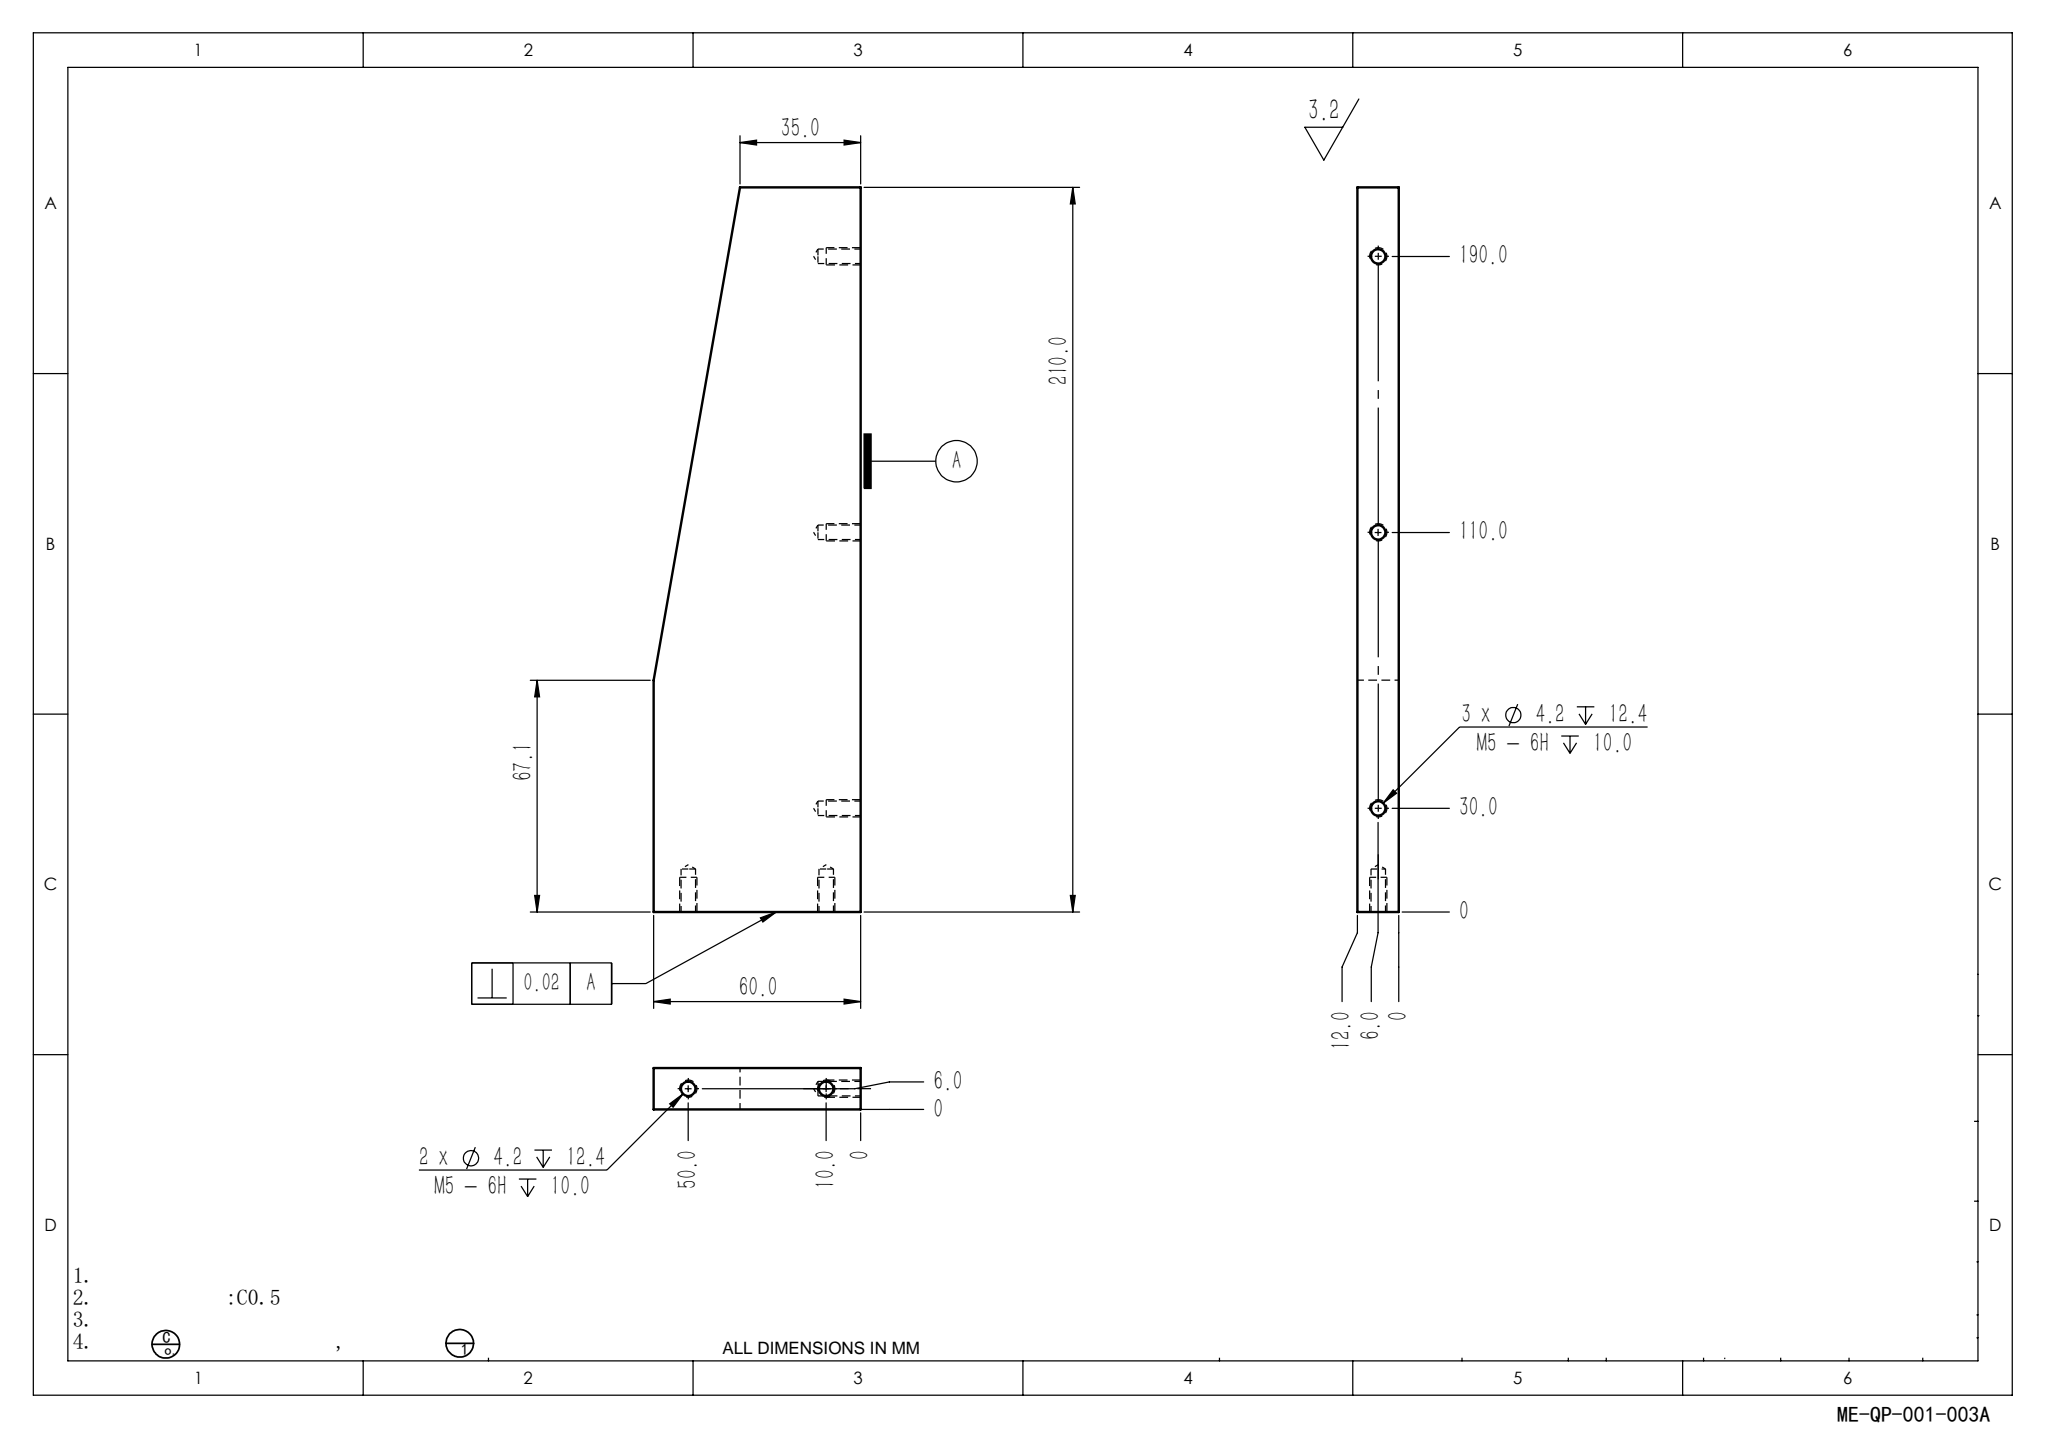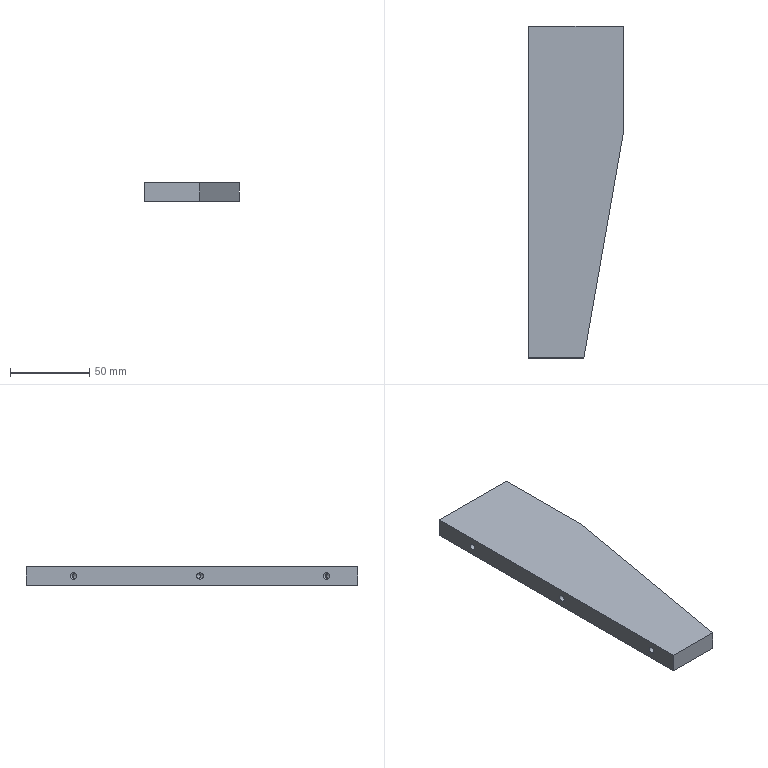Part | SolidWorks | mm | 1 solid | 27 faces | box 60 x 210 x 12 mm | volume 128883 mm3 | cylinder 10 | cone 10 | plane 7 | commonest cylinder face diameters 4.2 x10
STEP:
#1=CARTESIAN_POINT('',(-40.1,-85.,3.9));
#2=VERTEX_POINT('',#1);
#3=CARTESIAN_POINT('',(-40.1,-85.,8.1));
#4=VERTEX_POINT('',#3);
#5=CARTESIAN_POINT('',(-40.1,-85.,6.));
#6=DIRECTION('',(-1.,0.,0.));
#7=DIRECTION('',(0.,0.,1.));
#8=AXIS2_PLACEMENT_3D('',#5,#6,#7);
#9=CIRCLE('',#8,2.1);
#10=EDGE_CURVE('',#2,#4,#9,.T.);
#11=ORIENTED_EDGE('',*,*,#10,.F.);
#12=CARTESIAN_POINT('',(-52.5,-85.,3.9));
#13=VERTEX_POINT('',#12);
#14=CARTESIAN_POINT('',(-52.5,-85.,3.9));
#15=DIRECTION('',(-1.,0.,0.));
#16=VECTOR('',#15,1000.);
#17=LINE('',#14,#16);
#18=EDGE_CURVE('',#2,#13,#17,.T.);
#19=ORIENTED_EDGE('',*,*,#18,.T.);
#20=CARTESIAN_POINT('',(-52.5,-85.,8.1));
#21=VERTEX_POINT('',#20);
#22=CARTESIAN_POINT('',(-52.5,-85.,6.));
#23=DIRECTION('',(-1.,0.,0.));
#24=DIRECTION('',(0.,0.,1.));
#25=AXIS2_PLACEMENT_3D('',#22,#23,#24);
#26=CIRCLE('',#25,2.1);
#27=EDGE_CURVE('',#13,#21,#26,.T.);
#28=ORIENTED_EDGE('',*,*,#27,.T.);
#29=CARTESIAN_POINT('',(-52.5,-85.,8.1));
#30=DIRECTION('',(-1.,0.,0.));
#31=VECTOR('',#30,1000.);
#32=LINE('',#29,#31);
#33=EDGE_CURVE('',#4,#21,#32,.T.);
#34=ORIENTED_EDGE('',*,*,#33,.F.);
#35=EDGE_LOOP('',(#11,#19,#28,#34));
#36=FACE_OUTER_BOUND('',#35,.T.);
#37=CARTESIAN_POINT('',(-52.5,-85.,6.));
#38=DIRECTION('',(-1.,0.,0.));
#39=DIRECTION('',(0.,0.,1.));
#40=AXIS2_PLACEMENT_3D('',#37,#38,#39);
#41=CYLINDRICAL_SURFACE('',#40,2.1);
#42=ADVANCED_FACE('',(#36),#41,.F.);
#43=CARTESIAN_POINT('',(-38.838,-85.,6.));
#44=VERTEX_POINT('',#43);
#45=CARTESIAN_POINT('',(-40.1,-85.,8.1));
#46=DIRECTION('',(-0.515,0.,0.8572));
#47=VECTOR('',#46,1000.);
#48=LINE('',#45,#47);
#49=EDGE_CURVE('',#44,#4,#48,.T.);
#50=ORIENTED_EDGE('',*,*,#49,.F.);
#51=CARTESIAN_POINT('',(-40.1,-85.,3.9));
#52=DIRECTION('',(-0.515,0.,-0.8572));
#53=VECTOR('',#52,1000.);
#54=LINE('',#51,#53);
#55=EDGE_CURVE('',#44,#2,#54,.T.);
#56=ORIENTED_EDGE('',*,*,#55,.T.);
#57=ORIENTED_EDGE('',*,*,#10,.T.);
#58=EDGE_LOOP('',(#50,#56,#57));
#59=FACE_OUTER_BOUND('',#58,.T.);
#60=CARTESIAN_POINT('',(-40.1,-85.,6.));
#61=DIRECTION('',(-1.,0.,0.));
#62=DIRECTION('',(0.,0.,1.));
#63=AXIS2_PLACEMENT_3D('',#60,#61,#62);
#64=CONICAL_SURFACE('',#63,2.1,1.03);
#65=ADVANCED_FACE('',(#59),#64,.F.);
#66=CARTESIAN_POINT('',(-40.1,-5.,3.9));
#67=VERTEX_POINT('',#66);
#68=CARTESIAN_POINT('',(-40.1,-5.,8.1));
#69=VERTEX_POINT('',#68);
#70=CARTESIAN_POINT('',(-40.1,-5.,6.));
#71=DIRECTION('',(-1.,0.,0.));
#72=DIRECTION('',(0.,0.,1.));
#73=AXIS2_PLACEMENT_3D('',#70,#71,#72);
#74=CIRCLE('',#73,2.1);
#75=EDGE_CURVE('',#67,#69,#74,.T.);
#76=ORIENTED_EDGE('',*,*,#75,.F.);
#77=CARTESIAN_POINT('',(-52.5,-5.,3.9));
#78=VERTEX_POINT('',#77);
#79=CARTESIAN_POINT('',(-52.5,-5.,3.9));
#80=DIRECTION('',(-1.,0.,0.));
#81=VECTOR('',#80,1000.);
#82=LINE('',#79,#81);
#83=EDGE_CURVE('',#67,#78,#82,.T.);
#84=ORIENTED_EDGE('',*,*,#83,.T.);
#85=CARTESIAN_POINT('',(-52.5,-5.,8.1));
#86=VERTEX_POINT('',#85);
#87=CARTESIAN_POINT('',(-52.5,-5.,6.));
#88=DIRECTION('',(-1.,0.,0.));
#89=DIRECTION('',(0.,0.,1.));
#90=AXIS2_PLACEMENT_3D('',#87,#88,#89);
#91=CIRCLE('',#90,2.1);
#92=EDGE_CURVE('',#78,#86,#91,.T.);
#93=ORIENTED_EDGE('',*,*,#92,.T.);
#94=CARTESIAN_POINT('',(-52.5,-5.,8.1));
#95=DIRECTION('',(-1.,0.,0.));
#96=VECTOR('',#95,1000.);
#97=LINE('',#94,#96);
#98=EDGE_CURVE('',#69,#86,#97,.T.);
#99=ORIENTED_EDGE('',*,*,#98,.F.);
#100=EDGE_LOOP('',(#76,#84,#93,#99));
#101=FACE_OUTER_BOUND('',#100,.T.);
#102=CARTESIAN_POINT('',(-52.5,-5.,6.));
#103=DIRECTION('',(-1.,0.,0.));
#104=DIRECTION('',(0.,0.,1.));
#105=AXIS2_PLACEMENT_3D('',#102,#103,#104);
#106=CYLINDRICAL_SURFACE('',#105,2.1);
#107=ADVANCED_FACE('',(#101),#106,.F.);
#108=CARTESIAN_POINT('',(-38.838,-5.,6.));
#109=VERTEX_POINT('',#108);
#110=CARTESIAN_POINT('',(-40.1,-5.,8.1));
#111=DIRECTION('',(-0.515,0.,0.8572));
#112=VECTOR('',#111,1000.);
#113=LINE('',#110,#112);
#114=EDGE_CURVE('',#109,#69,#113,.T.);
#115=ORIENTED_EDGE('',*,*,#114,.F.);
#116=CARTESIAN_POINT('',(-40.1,-5.,3.9));
#117=DIRECTION('',(-0.515,0.,-0.8572));
#118=VECTOR('',#117,1000.);
#119=LINE('',#116,#118);
#120=EDGE_CURVE('',#109,#67,#119,.T.);
#121=ORIENTED_EDGE('',*,*,#120,.T.);
#122=ORIENTED_EDGE('',*,*,#75,.T.);
#123=EDGE_LOOP('',(#115,#121,#122));
#124=FACE_OUTER_BOUND('',#123,.T.);
#125=CARTESIAN_POINT('',(-40.1,-5.,6.));
#126=DIRECTION('',(-1.,0.,0.));
#127=DIRECTION('',(0.,0.,1.));
#128=AXIS2_PLACEMENT_3D('',#125,#126,#127);
#129=CONICAL_SURFACE('',#128,2.1,1.03);
#130=ADVANCED_FACE('',(#124),#129,.F.);
#131=CARTESIAN_POINT('',(-40.1,75.,3.9));
#132=VERTEX_POINT('',#131);
#133=CARTESIAN_POINT('',(-40.1,75.,8.1));
#134=VERTEX_POINT('',#133);
#135=CARTESIAN_POINT('',(-40.1,75.,6.));
#136=DIRECTION('',(-1.,0.,0.));
#137=DIRECTION('',(0.,0.,1.));
#138=AXIS2_PLACEMENT_3D('',#135,#136,#137);
#139=CIRCLE('',#138,2.1);
#140=EDGE_CURVE('',#132,#134,#139,.T.);
#141=ORIENTED_EDGE('',*,*,#140,.F.);
#142=CARTESIAN_POINT('',(-52.5,75.,3.9));
#143=VERTEX_POINT('',#142);
#144=CARTESIAN_POINT('',(-52.5,75.,3.9));
#145=DIRECTION('',(-1.,0.,0.));
#146=VECTOR('',#145,1000.);
#147=LINE('',#144,#146);
#148=EDGE_CURVE('',#132,#143,#147,.T.);
#149=ORIENTED_EDGE('',*,*,#148,.T.);
#150=CARTESIAN_POINT('',(-52.5,75.,8.1));
#151=VERTEX_POINT('',#150);
#152=CARTESIAN_POINT('',(-52.5,75.,6.));
#153=DIRECTION('',(-1.,0.,0.));
#154=DIRECTION('',(0.,0.,1.));
#155=AXIS2_PLACEMENT_3D('',#152,#153,#154);
#156=CIRCLE('',#155,2.1);
#157=EDGE_CURVE('',#143,#151,#156,.T.);
#158=ORIENTED_EDGE('',*,*,#157,.T.);
#159=CARTESIAN_POINT('',(-52.5,75.,8.1));
#160=DIRECTION('',(-1.,0.,0.));
#161=VECTOR('',#160,1000.);
#162=LINE('',#159,#161);
#163=EDGE_CURVE('',#134,#151,#162,.T.);
#164=ORIENTED_EDGE('',*,*,#163,.F.);
#165=EDGE_LOOP('',(#141,#149,#158,#164));
#166=FACE_OUTER_BOUND('',#165,.T.);
#167=CARTESIAN_POINT('',(-52.5,75.,6.));
#168=DIRECTION('',(-1.,0.,0.));
#169=DIRECTION('',(0.,0.,1.));
#170=AXIS2_PLACEMENT_3D('',#167,#168,#169);
#171=CYLINDRICAL_SURFACE('',#170,2.1);
#172=ADVANCED_FACE('',(#166),#171,.F.);
#173=CARTESIAN_POINT('',(-38.838,75.,6.));
#174=VERTEX_POINT('',#173);
#175=CARTESIAN_POINT('',(-40.1,75.,8.1));
#176=DIRECTION('',(-0.515,0.,0.8572));
#177=VECTOR('',#176,1000.);
#178=LINE('',#175,#177);
#179=EDGE_CURVE('',#174,#134,#178,.T.);
#180=ORIENTED_EDGE('',*,*,#179,.F.);
#181=CARTESIAN_POINT('',(-40.1,75.,3.9));
#182=DIRECTION('',(-0.515,0.,-0.8572));
#183=VECTOR('',#182,1000.);
#184=LINE('',#181,#183);
#185=EDGE_CURVE('',#174,#132,#184,.T.);
#186=ORIENTED_EDGE('',*,*,#185,.T.);
#187=ORIENTED_EDGE('',*,*,#140,.T.);
#188=EDGE_LOOP('',(#180,#186,#187));
#189=FACE_OUTER_BOUND('',#188,.T.);
#190=CARTESIAN_POINT('',(-40.1,75.,6.));
#191=DIRECTION('',(-1.,0.,0.));
#192=DIRECTION('',(0.,0.,1.));
#193=AXIS2_PLACEMENT_3D('',#190,#191,#192);
#194=CONICAL_SURFACE('',#193,2.1,1.03);
#195=ADVANCED_FACE('',(#189),#194,.F.);
#196=CARTESIAN_POINT('',(-42.5,92.6,3.9));
#197=VERTEX_POINT('',#196);
#198=CARTESIAN_POINT('',(-42.5,92.6,8.1));
#199=VERTEX_POINT('',#198);
#200=CARTESIAN_POINT('',(-42.5,92.6,6.));
#201=DIRECTION('',(0.,1.,0.));
#202=DIRECTION('',(0.,0.,1.));
#203=AXIS2_PLACEMENT_3D('',#200,#201,#202);
#204=CIRCLE('',#203,2.1);
#205=EDGE_CURVE('',#197,#199,#204,.T.);
#206=ORIENTED_EDGE('',*,*,#205,.F.);
#207=CARTESIAN_POINT('',(-42.5,105.,3.9));
#208=VERTEX_POINT('',#207);
#209=CARTESIAN_POINT('',(-42.5,105.,3.9));
#210=DIRECTION('',(0.,1.,0.));
#211=VECTOR('',#210,1000.);
#212=LINE('',#209,#211);
#213=EDGE_CURVE('',#197,#208,#212,.T.);
#214=ORIENTED_EDGE('',*,*,#213,.T.);
#215=CARTESIAN_POINT('',(-42.5,105.,8.1));
#216=VERTEX_POINT('',#215);
#217=CARTESIAN_POINT('',(-42.5,105.,6.));
#218=DIRECTION('',(0.,1.,0.));
#219=DIRECTION('',(0.,0.,1.));
#220=AXIS2_PLACEMENT_3D('',#217,#218,#219);
#221=CIRCLE('',#220,2.1);
#222=EDGE_CURVE('',#208,#216,#221,.T.);
#223=ORIENTED_EDGE('',*,*,#222,.T.);
#224=CARTESIAN_POINT('',(-42.5,105.,8.1));
#225=DIRECTION('',(0.,1.,0.));
#226=VECTOR('',#225,1000.);
#227=LINE('',#224,#226);
#228=EDGE_CURVE('',#199,#216,#227,.T.);
#229=ORIENTED_EDGE('',*,*,#228,.F.);
#230=EDGE_LOOP('',(#206,#214,#223,#229));
#231=FACE_OUTER_BOUND('',#230,.T.);
#232=CARTESIAN_POINT('',(-42.5,105.,6.));
#233=DIRECTION('',(0.,1.,0.));
#234=DIRECTION('',(0.,0.,1.));
#235=AXIS2_PLACEMENT_3D('',#232,#233,#234);
#236=CYLINDRICAL_SURFACE('',#235,2.1);
#237=ADVANCED_FACE('',(#231),#236,.F.);
#238=CARTESIAN_POINT('',(-42.5,91.338,6.));
#239=VERTEX_POINT('',#238);
#240=CARTESIAN_POINT('',(-42.5,92.6,8.1));
#241=DIRECTION('',(0.,0.515,0.8572));
#242=VECTOR('',#241,1000.);
#243=LINE('',#240,#242);
#244=EDGE_CURVE('',#239,#199,#243,.T.);
#245=ORIENTED_EDGE('',*,*,#244,.F.);
#246=CARTESIAN_POINT('',(-42.5,92.6,3.9));
#247=DIRECTION('',(0.,0.515,-0.8572));
#248=VECTOR('',#247,1000.);
#249=LINE('',#246,#248);
#250=EDGE_CURVE('',#239,#197,#249,.T.);
#251=ORIENTED_EDGE('',*,*,#250,.T.);
#252=ORIENTED_EDGE('',*,*,#205,.T.);
#253=EDGE_LOOP('',(#245,#251,#252));
#254=FACE_OUTER_BOUND('',#253,.T.);
#255=CARTESIAN_POINT('',(-42.5,92.6,6.));
#256=DIRECTION('',(0.,1.,0.));
#257=DIRECTION('',(0.,0.,1.));
#258=AXIS2_PLACEMENT_3D('',#255,#256,#257);
#259=CONICAL_SURFACE('',#258,2.1,1.03);
#260=ADVANCED_FACE('',(#254),#259,.F.);
#261=CARTESIAN_POINT('',(-2.5,92.6,3.9));
#262=VERTEX_POINT('',#261);
#263=CARTESIAN_POINT('',(-2.5,92.6,8.1));
#264=VERTEX_POINT('',#263);
#265=CARTESIAN_POINT('',(-2.5,92.6,6.));
#266=DIRECTION('',(0.,1.,0.));
#267=DIRECTION('',(0.,0.,1.));
#268=AXIS2_PLACEMENT_3D('',#265,#266,#267);
#269=CIRCLE('',#268,2.1);
#270=EDGE_CURVE('',#262,#264,#269,.T.);
#271=ORIENTED_EDGE('',*,*,#270,.F.);
#272=CARTESIAN_POINT('',(-2.5,105.,3.9));
#273=VERTEX_POINT('',#272);
#274=CARTESIAN_POINT('',(-2.5,105.,3.9));
#275=DIRECTION('',(0.,1.,0.));
#276=VECTOR('',#275,1000.);
#277=LINE('',#274,#276);
#278=EDGE_CURVE('',#262,#273,#277,.T.);
#279=ORIENTED_EDGE('',*,*,#278,.T.);
#280=CARTESIAN_POINT('',(-2.5,105.,8.1));
#281=VERTEX_POINT('',#280);
#282=CARTESIAN_POINT('',(-2.5,105.,6.));
#283=DIRECTION('',(0.,1.,0.));
#284=DIRECTION('',(0.,0.,1.));
#285=AXIS2_PLACEMENT_3D('',#282,#283,#284);
#286=CIRCLE('',#285,2.1);
#287=EDGE_CURVE('',#273,#281,#286,.T.);
#288=ORIENTED_EDGE('',*,*,#287,.T.);
#289=CARTESIAN_POINT('',(-2.5,105.,8.1));
#290=DIRECTION('',(0.,1.,0.));
#291=VECTOR('',#290,1000.);
#292=LINE('',#289,#291);
#293=EDGE_CURVE('',#264,#281,#292,.T.);
#294=ORIENTED_EDGE('',*,*,#293,.F.);
#295=EDGE_LOOP('',(#271,#279,#288,#294));
#296=FACE_OUTER_BOUND('',#295,.T.);
#297=CARTESIAN_POINT('',(-2.5,105.,6.));
#298=DIRECTION('',(0.,1.,0.));
#299=DIRECTION('',(0.,0.,1.));
#300=AXIS2_PLACEMENT_3D('',#297,#298,#299);
#301=CYLINDRICAL_SURFACE('',#300,2.1);
#302=ADVANCED_FACE('',(#296),#301,.F.);
#303=CARTESIAN_POINT('',(-2.5,91.338,6.));
#304=VERTEX_POINT('',#303);
#305=CARTESIAN_POINT('',(-2.5,92.6,8.1));
#306=DIRECTION('',(0.,0.515,0.8572));
#307=VECTOR('',#306,1000.);
#308=LINE('',#305,#307);
#309=EDGE_CURVE('',#304,#264,#308,.T.);
#310=ORIENTED_EDGE('',*,*,#309,.F.);
#311=CARTESIAN_POINT('',(-2.5,92.6,3.9));
#312=DIRECTION('',(0.,0.515,-0.8572));
#313=VECTOR('',#312,1000.);
#314=LINE('',#311,#313);
#315=EDGE_CURVE('',#304,#262,#314,.T.);
#316=ORIENTED_EDGE('',*,*,#315,.T.);
#317=ORIENTED_EDGE('',*,*,#270,.T.);
#318=EDGE_LOOP('',(#310,#316,#317));
#319=FACE_OUTER_BOUND('',#318,.T.);
#320=CARTESIAN_POINT('',(-2.5,92.6,6.));
#321=DIRECTION('',(0.,1.,0.));
#322=DIRECTION('',(0.,0.,1.));
#323=AXIS2_PLACEMENT_3D('',#320,#321,#322);
#324=CONICAL_SURFACE('',#323,2.1,1.03);
#325=ADVANCED_FACE('',(#319),#324,.F.);
#326=CARTESIAN_POINT('',(-52.5,-85.,6.));
#327=DIRECTION('',(-1.,0.,0.));
#328=DIRECTION('',(0.,0.,1.));
#329=AXIS2_PLACEMENT_3D('',#326,#327,#328);
#330=CIRCLE('',#329,2.1);
#331=EDGE_CURVE('',#21,#13,#330,.T.);
#332=ORIENTED_EDGE('',*,*,#331,.F.);
#333=ORIENTED_EDGE('',*,*,#27,.F.);
#334=EDGE_LOOP('',(#332,#333));
#335=FACE_BOUND('',#334,.T.);
#336=CARTESIAN_POINT('',(-52.5,-5.,6.));
#337=DIRECTION('',(-1.,0.,0.));
#338=DIRECTION('',(0.,0.,1.));
#339=AXIS2_PLACEMENT_3D('',#336,#337,#338);
#340=CIRCLE('',#339,2.1);
#341=EDGE_CURVE('',#86,#78,#340,.T.);
#342=ORIENTED_EDGE('',*,*,#341,.F.);
#343=ORIENTED_EDGE('',*,*,#92,.F.);
#344=EDGE_LOOP('',(#342,#343));
#345=FACE_BOUND('',#344,.T.);
#346=CARTESIAN_POINT('',(-52.5,75.,6.));
#347=DIRECTION('',(-1.,0.,0.));
#348=DIRECTION('',(0.,0.,1.));
#349=AXIS2_PLACEMENT_3D('',#346,#347,#348);
#350=CIRCLE('',#349,2.1);
#351=EDGE_CURVE('',#151,#143,#350,.T.);
#352=ORIENTED_EDGE('',*,*,#351,.F.);
#353=ORIENTED_EDGE('',*,*,#157,.F.);
#354=EDGE_LOOP('',(#352,#353));
#355=FACE_BOUND('',#354,.T.);
#356=CARTESIAN_POINT('',(-52.5,105.,0.));
#357=VERTEX_POINT('',#356);
#358=CARTESIAN_POINT('',(-52.5,-105.,0.));
#359=VERTEX_POINT('',#358);
#360=CARTESIAN_POINT('',(-52.5,-105.,0.));
#361=DIRECTION('',(0.,-1.,0.));
#362=VECTOR('',#361,1000.);
#363=LINE('',#360,#362);
#364=EDGE_CURVE('',#357,#359,#363,.T.);
#365=ORIENTED_EDGE('',*,*,#364,.T.);
#366=CARTESIAN_POINT('',(-52.5,-105.,12.));
#367=VERTEX_POINT('',#366);
#368=CARTESIAN_POINT('',(-52.5,-105.,12.));
#369=DIRECTION('',(0.,0.,-1.));
#370=VECTOR('',#369,1000.);
#371=LINE('',#368,#370);
#372=EDGE_CURVE('',#367,#359,#371,.T.);
#373=ORIENTED_EDGE('',*,*,#372,.F.);
#374=CARTESIAN_POINT('',(-52.5,105.,12.));
#375=VERTEX_POINT('',#374);
#376=CARTESIAN_POINT('',(-52.5,-105.,12.));
#377=DIRECTION('',(0.,-1.,0.));
#378=VECTOR('',#377,1000.);
#379=LINE('',#376,#378);
#380=EDGE_CURVE('',#375,#367,#379,.T.);
#381=ORIENTED_EDGE('',*,*,#380,.F.);
#382=CARTESIAN_POINT('',(-52.5,105.,12.));
#383=DIRECTION('',(0.,0.,-1.));
#384=VECTOR('',#383,1000.);
#385=LINE('',#382,#384);
#386=EDGE_CURVE('',#375,#357,#385,.T.);
#387=ORIENTED_EDGE('',*,*,#386,.T.);
#388=EDGE_LOOP('',(#365,#373,#381,#387));
#389=FACE_OUTER_BOUND('',#388,.T.);
#390=CARTESIAN_POINT('',(-52.5,-105.,12.));
#391=DIRECTION('',(1.,0.,0.));
#392=DIRECTION('',(0.,0.,-1.));
#393=AXIS2_PLACEMENT_3D('',#390,#391,#392);
#394=PLANE('',#393);
#395=ADVANCED_FACE('',(#335,#345,#355,#389),#394,.F.);
#396=CARTESIAN_POINT('',(-17.5,-105.,0.));
#397=VERTEX_POINT('',#396);
#398=CARTESIAN_POINT('',(52.5,-105.,0.));
#399=DIRECTION('',(1.,0.,0.));
#400=VECTOR('',#399,1000.);
#401=LINE('',#398,#400);
#402=EDGE_CURVE('',#359,#397,#401,.T.);
#403=ORIENTED_EDGE('',*,*,#402,.T.);
#404=CARTESIAN_POINT('',(-17.5,-105.,12.));
#405=VERTEX_POINT('',#404);
#406=CARTESIAN_POINT('',(-17.5,-105.,12.));
#407=DIRECTION('',(0.,0.,1.));
#408=VECTOR('',#407,1000.);
#409=LINE('',#406,#408);
#410=EDGE_CURVE('',#397,#405,#409,.T.);
#411=ORIENTED_EDGE('',*,*,#410,.T.);
#412=CARTESIAN_POINT('',(52.5,-105.,12.));
#413=DIRECTION('',(1.,0.,0.));
#414=VECTOR('',#413,1000.);
#415=LINE('',#412,#414);
#416=EDGE_CURVE('',#367,#405,#415,.T.);
#417=ORIENTED_EDGE('',*,*,#416,.F.);
#418=ORIENTED_EDGE('',*,*,#372,.T.);
#419=EDGE_LOOP('',(#403,#411,#417,#418));
#420=FACE_OUTER_BOUND('',#419,.T.);
#421=CARTESIAN_POINT('',(52.5,-105.,12.));
#422=DIRECTION('',(-0.,1.,0.));
#423=DIRECTION('',(-1.,-0.,0.));
#424=AXIS2_PLACEMENT_3D('',#421,#422,#423);
#425=PLANE('',#424);
#426=ADVANCED_FACE('',(#420),#425,.F.);
#427=CARTESIAN_POINT('',(-42.5,105.,6.));
#428=DIRECTION('',(0.,1.,0.));
#429=DIRECTION('',(0.,0.,1.));
#430=AXIS2_PLACEMENT_3D('',#427,#428,#429);
#431=CIRCLE('',#430,2.1);
#432=EDGE_CURVE('',#216,#208,#431,.T.);
#433=ORIENTED_EDGE('',*,*,#432,.F.);
#434=ORIENTED_EDGE('',*,*,#222,.F.);
#435=EDGE_LOOP('',(#433,#434));
#436=FACE_BOUND('',#435,.T.);
#437=CARTESIAN_POINT('',(-2.5,105.,6.));
#438=DIRECTION('',(0.,1.,0.));
#439=DIRECTION('',(0.,0.,1.));
#440=AXIS2_PLACEMENT_3D('',#437,#438,#439);
#441=CIRCLE('',#440,2.1);
#442=EDGE_CURVE('',#281,#273,#441,.T.);
#443=ORIENTED_EDGE('',*,*,#442,.F.);
#444=ORIENTED_EDGE('',*,*,#287,.F.);
#445=EDGE_LOOP('',(#443,#444));
#446=FACE_BOUND('',#445,.T.);
#447=CARTESIAN_POINT('',(7.5,105.,12.));
#448=VERTEX_POINT('',#447);
#449=CARTESIAN_POINT('',(52.5,105.,12.));
#450=DIRECTION('',(-1.,0.,0.));
#451=VECTOR('',#450,1000.);
#452=LINE('',#449,#451);
#453=EDGE_CURVE('',#448,#375,#452,.T.);
#454=ORIENTED_EDGE('',*,*,#453,.F.);
#455=CARTESIAN_POINT('',(7.5,105.,0.));
#456=VERTEX_POINT('',#455);
#457=CARTESIAN_POINT('',(7.5,105.,12.));
#458=DIRECTION('',(0.,0.,-1.));
#459=VECTOR('',#458,1000.);
#460=LINE('',#457,#459);
#461=EDGE_CURVE('',#448,#456,#460,.T.);
#462=ORIENTED_EDGE('',*,*,#461,.T.);
#463=CARTESIAN_POINT('',(52.5,105.,0.));
#464=DIRECTION('',(-1.,0.,0.));
#465=VECTOR('',#464,1000.);
#466=LINE('',#463,#465);
#467=EDGE_CURVE('',#456,#357,#466,.T.);
#468=ORIENTED_EDGE('',*,*,#467,.T.);
#469=ORIENTED_EDGE('',*,*,#386,.F.);
#470=EDGE_LOOP('',(#454,#462,#468,#469));
#471=FACE_OUTER_BOUND('',#470,.T.);
#472=CARTESIAN_POINT('',(52.5,105.,12.));
#473=DIRECTION('',(0.,-1.,0.));
#474=DIRECTION('',(0.,0.,-1.));
#475=AXIS2_PLACEMENT_3D('',#472,#473,#474);
#476=PLANE('',#475);
#477=ADVANCED_FACE('',(#436,#446,#471),#476,.F.);
#478=CARTESIAN_POINT('',(7.5,37.857,12.));
#479=VERTEX_POINT('',#478);
#480=CARTESIAN_POINT('',(7.5,185.,12.));
#481=DIRECTION('',(0.,1.,0.));
#482=VECTOR('',#481,1000.);
#483=LINE('',#480,#482);
#484=EDGE_CURVE('',#479,#448,#483,.T.);
#485=ORIENTED_EDGE('',*,*,#484,.T.);
#486=ORIENTED_EDGE('',*,*,#453,.T.);
#487=ORIENTED_EDGE('',*,*,#380,.T.);
#488=ORIENTED_EDGE('',*,*,#416,.T.);
#489=CARTESIAN_POINT('',(0.849,-0.1486,12.));
#490=DIRECTION('',(0.1724,0.985,0.));
#491=VECTOR('',#490,1000.);
#492=LINE('',#489,#491);
#493=EDGE_CURVE('',#405,#479,#492,.T.);
#494=ORIENTED_EDGE('',*,*,#493,.T.);
#495=EDGE_LOOP('',(#485,#486,#487,#488,#494));
#496=FACE_OUTER_BOUND('',#495,.T.);
#497=CARTESIAN_POINT('',(0.,0.,12.));
#498=DIRECTION('',(0.,0.,1.));
#499=DIRECTION('',(1.,0.,0.));
#500=AXIS2_PLACEMENT_3D('',#497,#498,#499);
#501=PLANE('',#500);
#502=ADVANCED_FACE('',(#496),#501,.T.);
#503=ORIENTED_EDGE('',*,*,#467,.F.);
#504=CARTESIAN_POINT('',(7.5,37.857,0.));
#505=VERTEX_POINT('',#504);
#506=CARTESIAN_POINT('',(7.5,185.,0.));
#507=DIRECTION('',(0.,1.,0.));
#508=VECTOR('',#507,1000.);
#509=LINE('',#506,#508);
#510=EDGE_CURVE('',#505,#456,#509,.T.);
#511=ORIENTED_EDGE('',*,*,#510,.F.);
#512=CARTESIAN_POINT('',(52.5,295.,0.));
#513=DIRECTION('',(-0.1724,-0.985,0.));
#514=VECTOR('',#513,1000.);
#515=LINE('',#512,#514);
#516=EDGE_CURVE('',#505,#397,#515,.T.);
#517=ORIENTED_EDGE('',*,*,#516,.T.);
#518=ORIENTED_EDGE('',*,*,#402,.F.);
#519=ORIENTED_EDGE('',*,*,#364,.F.);
#520=EDGE_LOOP('',(#503,#511,#517,#518,#519));
#521=FACE_OUTER_BOUND('',#520,.T.);
#522=CARTESIAN_POINT('',(0.,0.,0.));
#523=DIRECTION('',(0.,0.,1.));
#524=DIRECTION('',(1.,0.,0.));
#525=AXIS2_PLACEMENT_3D('',#522,#523,#524);
#526=PLANE('',#525);
#527=ADVANCED_FACE('',(#521),#526,.F.);
#528=CARTESIAN_POINT('',(7.5,37.857,12.));
#529=DIRECTION('',(0.,0.,-1.));
#530=VECTOR('',#529,1000.);
#531=LINE('',#528,#530);
#532=EDGE_CURVE('',#479,#505,#531,.T.);
#533=ORIENTED_EDGE('',*,*,#532,.F.);
#534=ORIENTED_EDGE('',*,*,#493,.F.);
#535=ORIENTED_EDGE('',*,*,#410,.F.);
#536=ORIENTED_EDGE('',*,*,#516,.F.);
#537=EDGE_LOOP('',(#533,#534,#535,#536));
#538=FACE_OUTER_BOUND('',#537,.T.);
#539=CARTESIAN_POINT('',(52.5,295.,12.));
#540=DIRECTION('',(-0.985,0.1724,0.));
#541=DIRECTION('',(0.,0.,-1.));
#542=AXIS2_PLACEMENT_3D('',#539,#540,#541);
#543=PLANE('',#542);
#544=ADVANCED_FACE('',(#538),#543,.F.);
#545=ORIENTED_EDGE('',*,*,#315,.F.);
#546=ORIENTED_EDGE('',*,*,#309,.T.);
#547=CARTESIAN_POINT('',(-2.5,92.6,6.));
#548=DIRECTION('',(0.,1.,0.));
#549=DIRECTION('',(0.,0.,1.));
#550=AXIS2_PLACEMENT_3D('',#547,#548,#549);
#551=CIRCLE('',#550,2.1);
#552=EDGE_CURVE('',#264,#262,#551,.T.);
#553=ORIENTED_EDGE('',*,*,#552,.T.);
#554=EDGE_LOOP('',(#545,#546,#553));
#555=FACE_OUTER_BOUND('',#554,.T.);
#556=CARTESIAN_POINT('',(-2.5,92.6,6.));
#557=DIRECTION('',(0.,1.,0.));
#558=DIRECTION('',(0.,0.,1.));
#559=AXIS2_PLACEMENT_3D('',#556,#557,#558);
#560=CONICAL_SURFACE('',#559,2.1,1.03);
#561=ADVANCED_FACE('',(#555),#560,.F.);
#562=ORIENTED_EDGE('',*,*,#278,.F.);
#563=ORIENTED_EDGE('',*,*,#552,.F.);
#564=ORIENTED_EDGE('',*,*,#293,.T.);
#565=ORIENTED_EDGE('',*,*,#442,.T.);
#566=EDGE_LOOP('',(#562,#563,#564,#565));
#567=FACE_OUTER_BOUND('',#566,.T.);
#568=CARTESIAN_POINT('',(-2.5,105.,6.));
#569=DIRECTION('',(0.,1.,0.));
#570=DIRECTION('',(0.,0.,1.));
#571=AXIS2_PLACEMENT_3D('',#568,#569,#570);
#572=CYLINDRICAL_SURFACE('',#571,2.1);
#573=ADVANCED_FACE('',(#567),#572,.F.);
#574=ORIENTED_EDGE('',*,*,#250,.F.);
#575=ORIENTED_EDGE('',*,*,#244,.T.);
#576=CARTESIAN_POINT('',(-42.5,92.6,6.));
#577=DIRECTION('',(0.,1.,0.));
#578=DIRECTION('',(0.,0.,1.));
#579=AXIS2_PLACEMENT_3D('',#576,#577,#578);
#580=CIRCLE('',#579,2.1);
#581=EDGE_CURVE('',#199,#197,#580,.T.);
#582=ORIENTED_EDGE('',*,*,#581,.T.);
#583=EDGE_LOOP('',(#574,#575,#582));
#584=FACE_OUTER_BOUND('',#583,.T.);
#585=CARTESIAN_POINT('',(-42.5,92.6,6.));
#586=DIRECTION('',(0.,1.,0.));
#587=DIRECTION('',(0.,0.,1.));
#588=AXIS2_PLACEMENT_3D('',#585,#586,#587);
#589=CONICAL_SURFACE('',#588,2.1,1.03);
#590=ADVANCED_FACE('',(#584),#589,.F.);
#591=ORIENTED_EDGE('',*,*,#213,.F.);
#592=ORIENTED_EDGE('',*,*,#581,.F.);
#593=ORIENTED_EDGE('',*,*,#228,.T.);
#594=ORIENTED_EDGE('',*,*,#432,.T.);
#595=EDGE_LOOP('',(#591,#592,#593,#594));
#596=FACE_OUTER_BOUND('',#595,.T.);
#597=CARTESIAN_POINT('',(-42.5,105.,6.));
#598=DIRECTION('',(0.,1.,0.));
#599=DIRECTION('',(0.,0.,1.));
#600=AXIS2_PLACEMENT_3D('',#597,#598,#599);
#601=CYLINDRICAL_SURFACE('',#600,2.1);
#602=ADVANCED_FACE('',(#596),#601,.F.);
#603=ORIENTED_EDGE('',*,*,#185,.F.);
#604=ORIENTED_EDGE('',*,*,#179,.T.);
#605=CARTESIAN_POINT('',(-40.1,75.,6.));
#606=DIRECTION('',(-1.,0.,0.));
#607=DIRECTION('',(0.,0.,1.));
#608=AXIS2_PLACEMENT_3D('',#605,#606,#607);
#609=CIRCLE('',#608,2.1);
#610=EDGE_CURVE('',#134,#132,#609,.T.);
#611=ORIENTED_EDGE('',*,*,#610,.T.);
#612=EDGE_LOOP('',(#603,#604,#611));
#613=FACE_OUTER_BOUND('',#612,.T.);
#614=CARTESIAN_POINT('',(-40.1,75.,6.));
#615=DIRECTION('',(-1.,0.,0.));
#616=DIRECTION('',(0.,0.,1.));
#617=AXIS2_PLACEMENT_3D('',#614,#615,#616);
#618=CONICAL_SURFACE('',#617,2.1,1.03);
#619=ADVANCED_FACE('',(#613),#618,.F.);
#620=ORIENTED_EDGE('',*,*,#148,.F.);
#621=ORIENTED_EDGE('',*,*,#610,.F.);
#622=ORIENTED_EDGE('',*,*,#163,.T.);
#623=ORIENTED_EDGE('',*,*,#351,.T.);
#624=EDGE_LOOP('',(#620,#621,#622,#623));
#625=FACE_OUTER_BOUND('',#624,.T.);
#626=CARTESIAN_POINT('',(-52.5,75.,6.));
#627=DIRECTION('',(-1.,0.,0.));
#628=DIRECTION('',(0.,0.,1.));
#629=AXIS2_PLACEMENT_3D('',#626,#627,#628);
#630=CYLINDRICAL_SURFACE('',#629,2.1);
#631=ADVANCED_FACE('',(#625),#630,.F.);
#632=ORIENTED_EDGE('',*,*,#120,.F.);
#633=ORIENTED_EDGE('',*,*,#114,.T.);
#634=CARTESIAN_POINT('',(-40.1,-5.,6.));
#635=DIRECTION('',(-1.,0.,0.));
#636=DIRECTION('',(0.,0.,1.));
#637=AXIS2_PLACEMENT_3D('',#634,#635,#636);
#638=CIRCLE('',#637,2.1);
#639=EDGE_CURVE('',#69,#67,#638,.T.);
#640=ORIENTED_EDGE('',*,*,#639,.T.);
#641=EDGE_LOOP('',(#632,#633,#640));
#642=FACE_OUTER_BOUND('',#641,.T.);
#643=CARTESIAN_POINT('',(-40.1,-5.,6.));
#644=DIRECTION('',(-1.,0.,0.));
#645=DIRECTION('',(0.,0.,1.));
#646=AXIS2_PLACEMENT_3D('',#643,#644,#645);
#647=CONICAL_SURFACE('',#646,2.1,1.03);
#648=ADVANCED_FACE('',(#642),#647,.F.);
#649=ORIENTED_EDGE('',*,*,#83,.F.);
#650=ORIENTED_EDGE('',*,*,#639,.F.);
#651=ORIENTED_EDGE('',*,*,#98,.T.);
#652=ORIENTED_EDGE('',*,*,#341,.T.);
#653=EDGE_LOOP('',(#649,#650,#651,#652));
#654=FACE_OUTER_BOUND('',#653,.T.);
#655=CARTESIAN_POINT('',(-52.5,-5.,6.));
#656=DIRECTION('',(-1.,0.,0.));
#657=DIRECTION('',(0.,0.,1.));
#658=AXIS2_PLACEMENT_3D('',#655,#656,#657);
#659=CYLINDRICAL_SURFACE('',#658,2.1);
#660=ADVANCED_FACE('',(#654),#659,.F.);
#661=ORIENTED_EDGE('',*,*,#55,.F.);
#662=ORIENTED_EDGE('',*,*,#49,.T.);
#663=CARTESIAN_POINT('',(-40.1,-85.,6.));
#664=DIRECTION('',(-1.,0.,0.));
#665=DIRECTION('',(0.,0.,1.));
#666=AXIS2_PLACEMENT_3D('',#663,#664,#665);
#667=CIRCLE('',#666,2.1);
#668=EDGE_CURVE('',#4,#2,#667,.T.);
#669=ORIENTED_EDGE('',*,*,#668,.T.);
#670=EDGE_LOOP('',(#661,#662,#669));
#671=FACE_OUTER_BOUND('',#670,.T.);
#672=CARTESIAN_POINT('',(-40.1,-85.,6.));
#673=DIRECTION('',(-1.,0.,0.));
#674=DIRECTION('',(0.,0.,1.));
#675=AXIS2_PLACEMENT_3D('',#672,#673,#674);
#676=CONICAL_SURFACE('',#675,2.1,1.03);
#677=ADVANCED_FACE('',(#671),#676,.F.);
#678=ORIENTED_EDGE('',*,*,#18,.F.);
#679=ORIENTED_EDGE('',*,*,#668,.F.);
#680=ORIENTED_EDGE('',*,*,#33,.T.);
#681=ORIENTED_EDGE('',*,*,#331,.T.);
#682=EDGE_LOOP('',(#678,#679,#680,#681));
#683=FACE_OUTER_BOUND('',#682,.T.);
#684=CARTESIAN_POINT('',(-52.5,-85.,6.));
#685=DIRECTION('',(-1.,0.,0.));
#686=DIRECTION('',(0.,0.,1.));
#687=AXIS2_PLACEMENT_3D('',#684,#685,#686);
#688=CYLINDRICAL_SURFACE('',#687,2.1);
#689=ADVANCED_FACE('',(#683),#688,.F.);
#690=ORIENTED_EDGE('',*,*,#484,.F.);
#691=ORIENTED_EDGE('',*,*,#532,.T.);
#692=ORIENTED_EDGE('',*,*,#510,.T.);
#693=ORIENTED_EDGE('',*,*,#461,.F.);
#694=EDGE_LOOP('',(#690,#691,#692,#693));
#695=FACE_OUTER_BOUND('',#694,.T.);
#696=CARTESIAN_POINT('',(7.5,185.,12.));
#697=DIRECTION('',(-1.,0.,0.));
#698=DIRECTION('',(0.,0.,1.));
#699=AXIS2_PLACEMENT_3D('',#696,#697,#698);
#700=PLANE('',#699);
#701=ADVANCED_FACE('',(#695),#700,.F.);
#702=CLOSED_SHELL('',(#42,#65,#107,#130,#172,#195,#237,#260,#302,#325,#395,#426,#477,#502,#527,#544,#561,#573,#590,#602,#619,#631,#648,#660,#677,#689,#701));
#703=MANIFOLD_SOLID_BREP('',#702);
#704=CARTESIAN_POINT('',(0.,0.,0.));
#705=DIRECTION('',(0.,0.,1.));
#706=DIRECTION('',(1.,0.,0.));
#707=AXIS2_PLACEMENT_3D('',#704,#705,#706);
#708=(LENGTH_UNIT()NAMED_UNIT(*)SI_UNIT(.MILLI.,.METRE.));
#709=UNCERTAINTY_MEASURE_WITH_UNIT(LENGTH_MEASURE(0.00001),#708,'','');
#710=(NAMED_UNIT(*)PLANE_ANGLE_UNIT()SI_UNIT($,.RADIAN.));
#711=(NAMED_UNIT(*)SI_UNIT($,.STERADIAN.)SOLID_ANGLE_UNIT());
#712=(GEOMETRIC_REPRESENTATION_CONTEXT(3)GLOBAL_UNCERTAINTY_ASSIGNED_CONTEXT((#709))GLOBAL_UNIT_ASSIGNED_CONTEXT((#708,#710,#711))REPRESENTATION_CONTEXT('',''));
#713=ADVANCED_BREP_SHAPE_REPRESENTATION('',(#703,#707),#712);